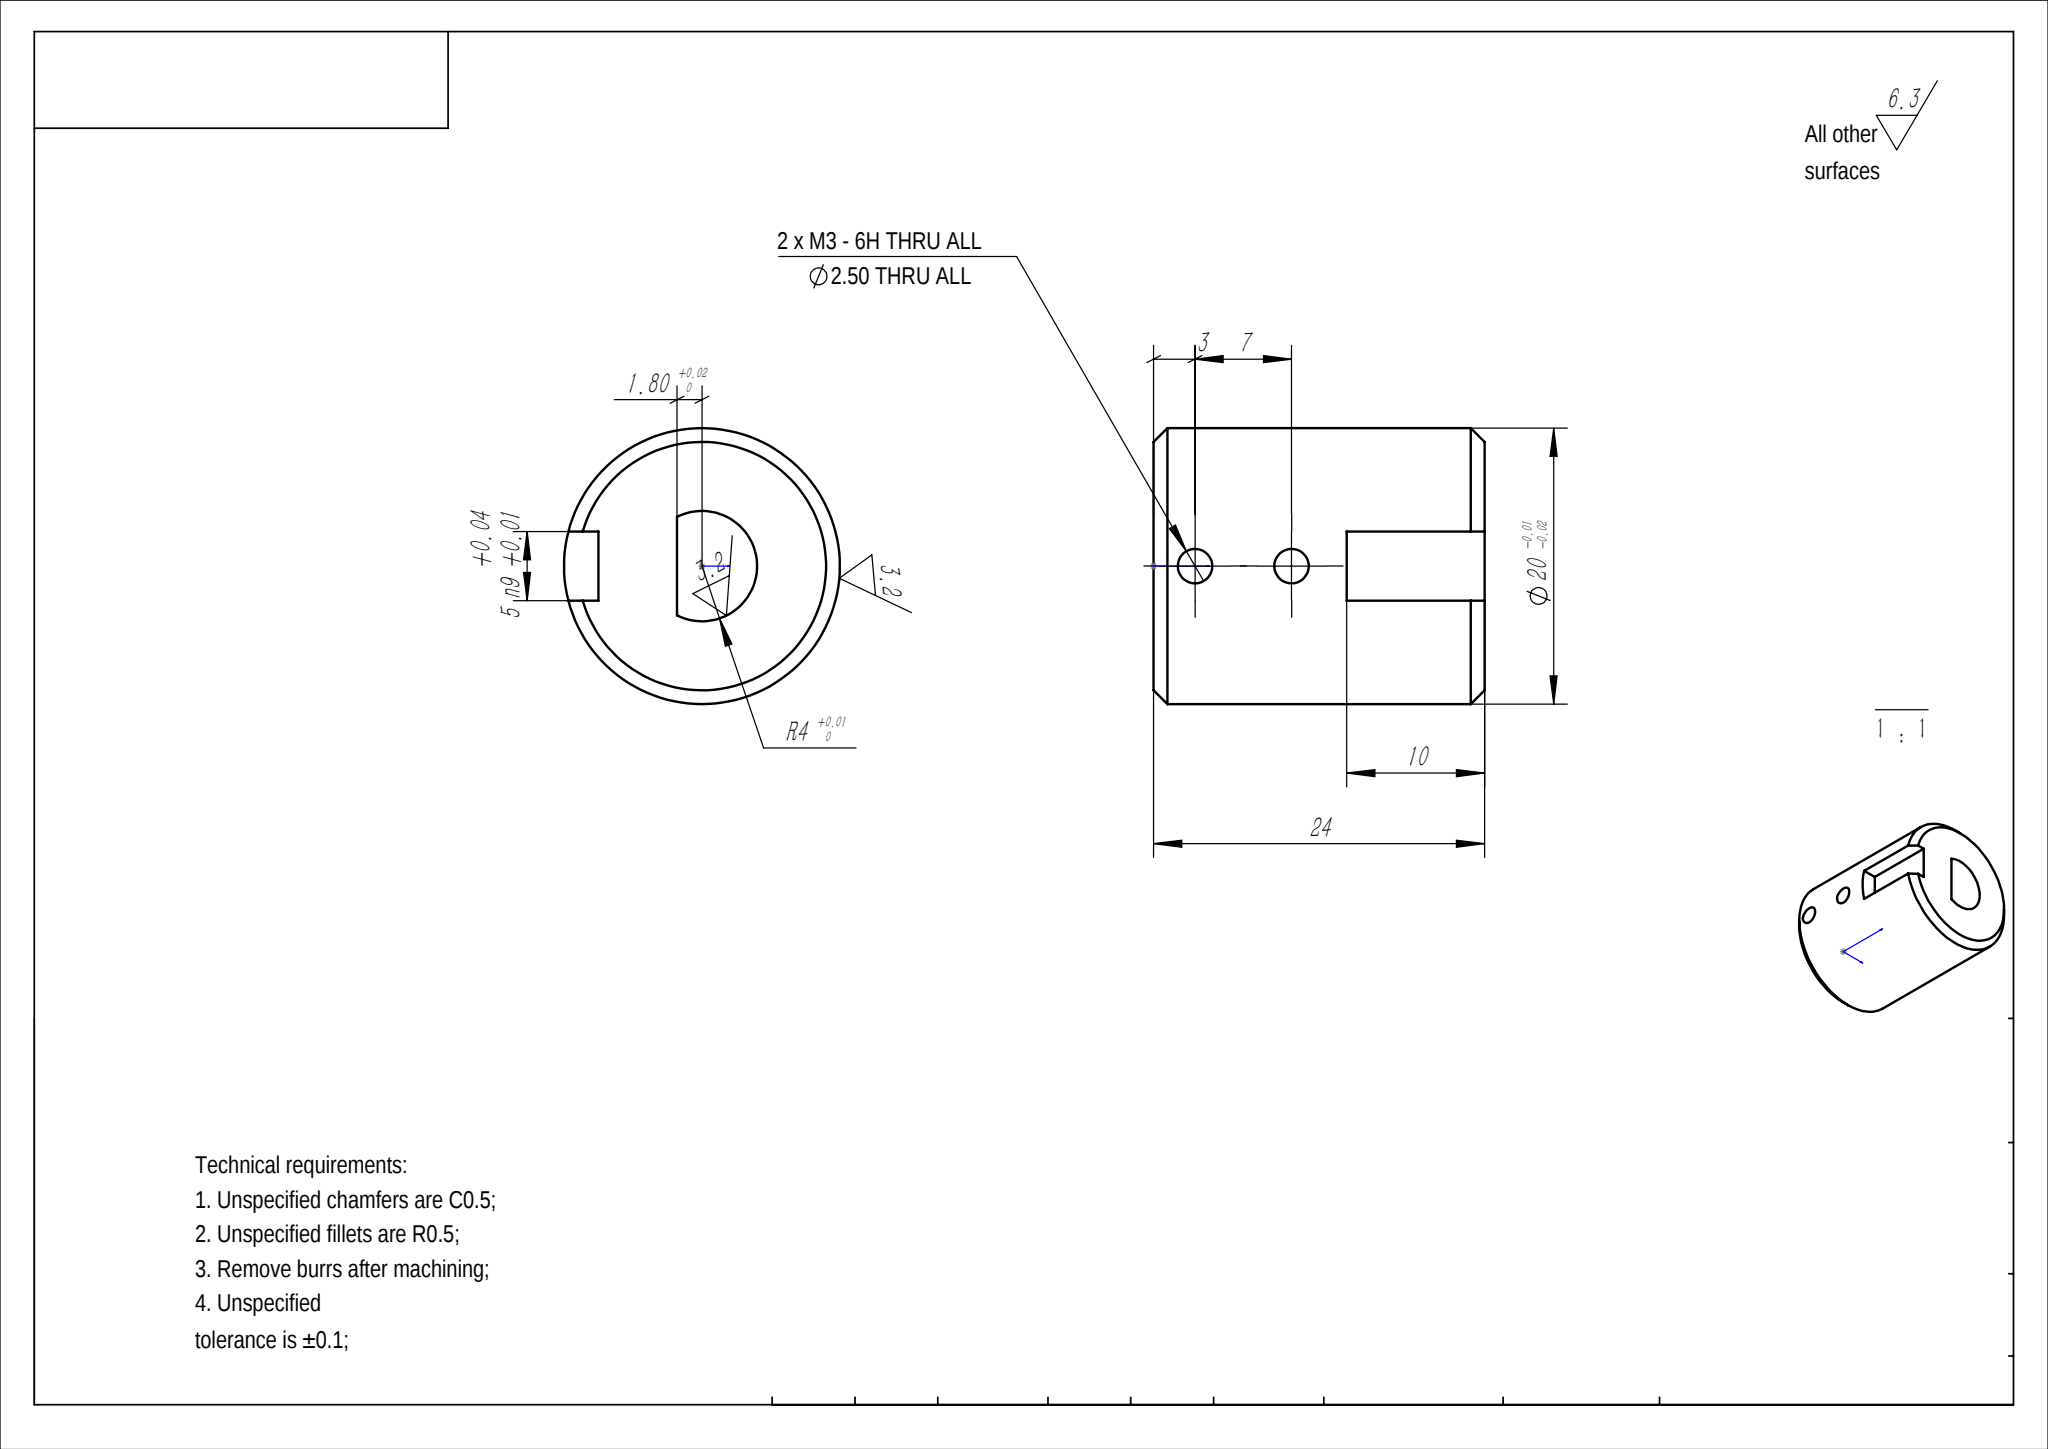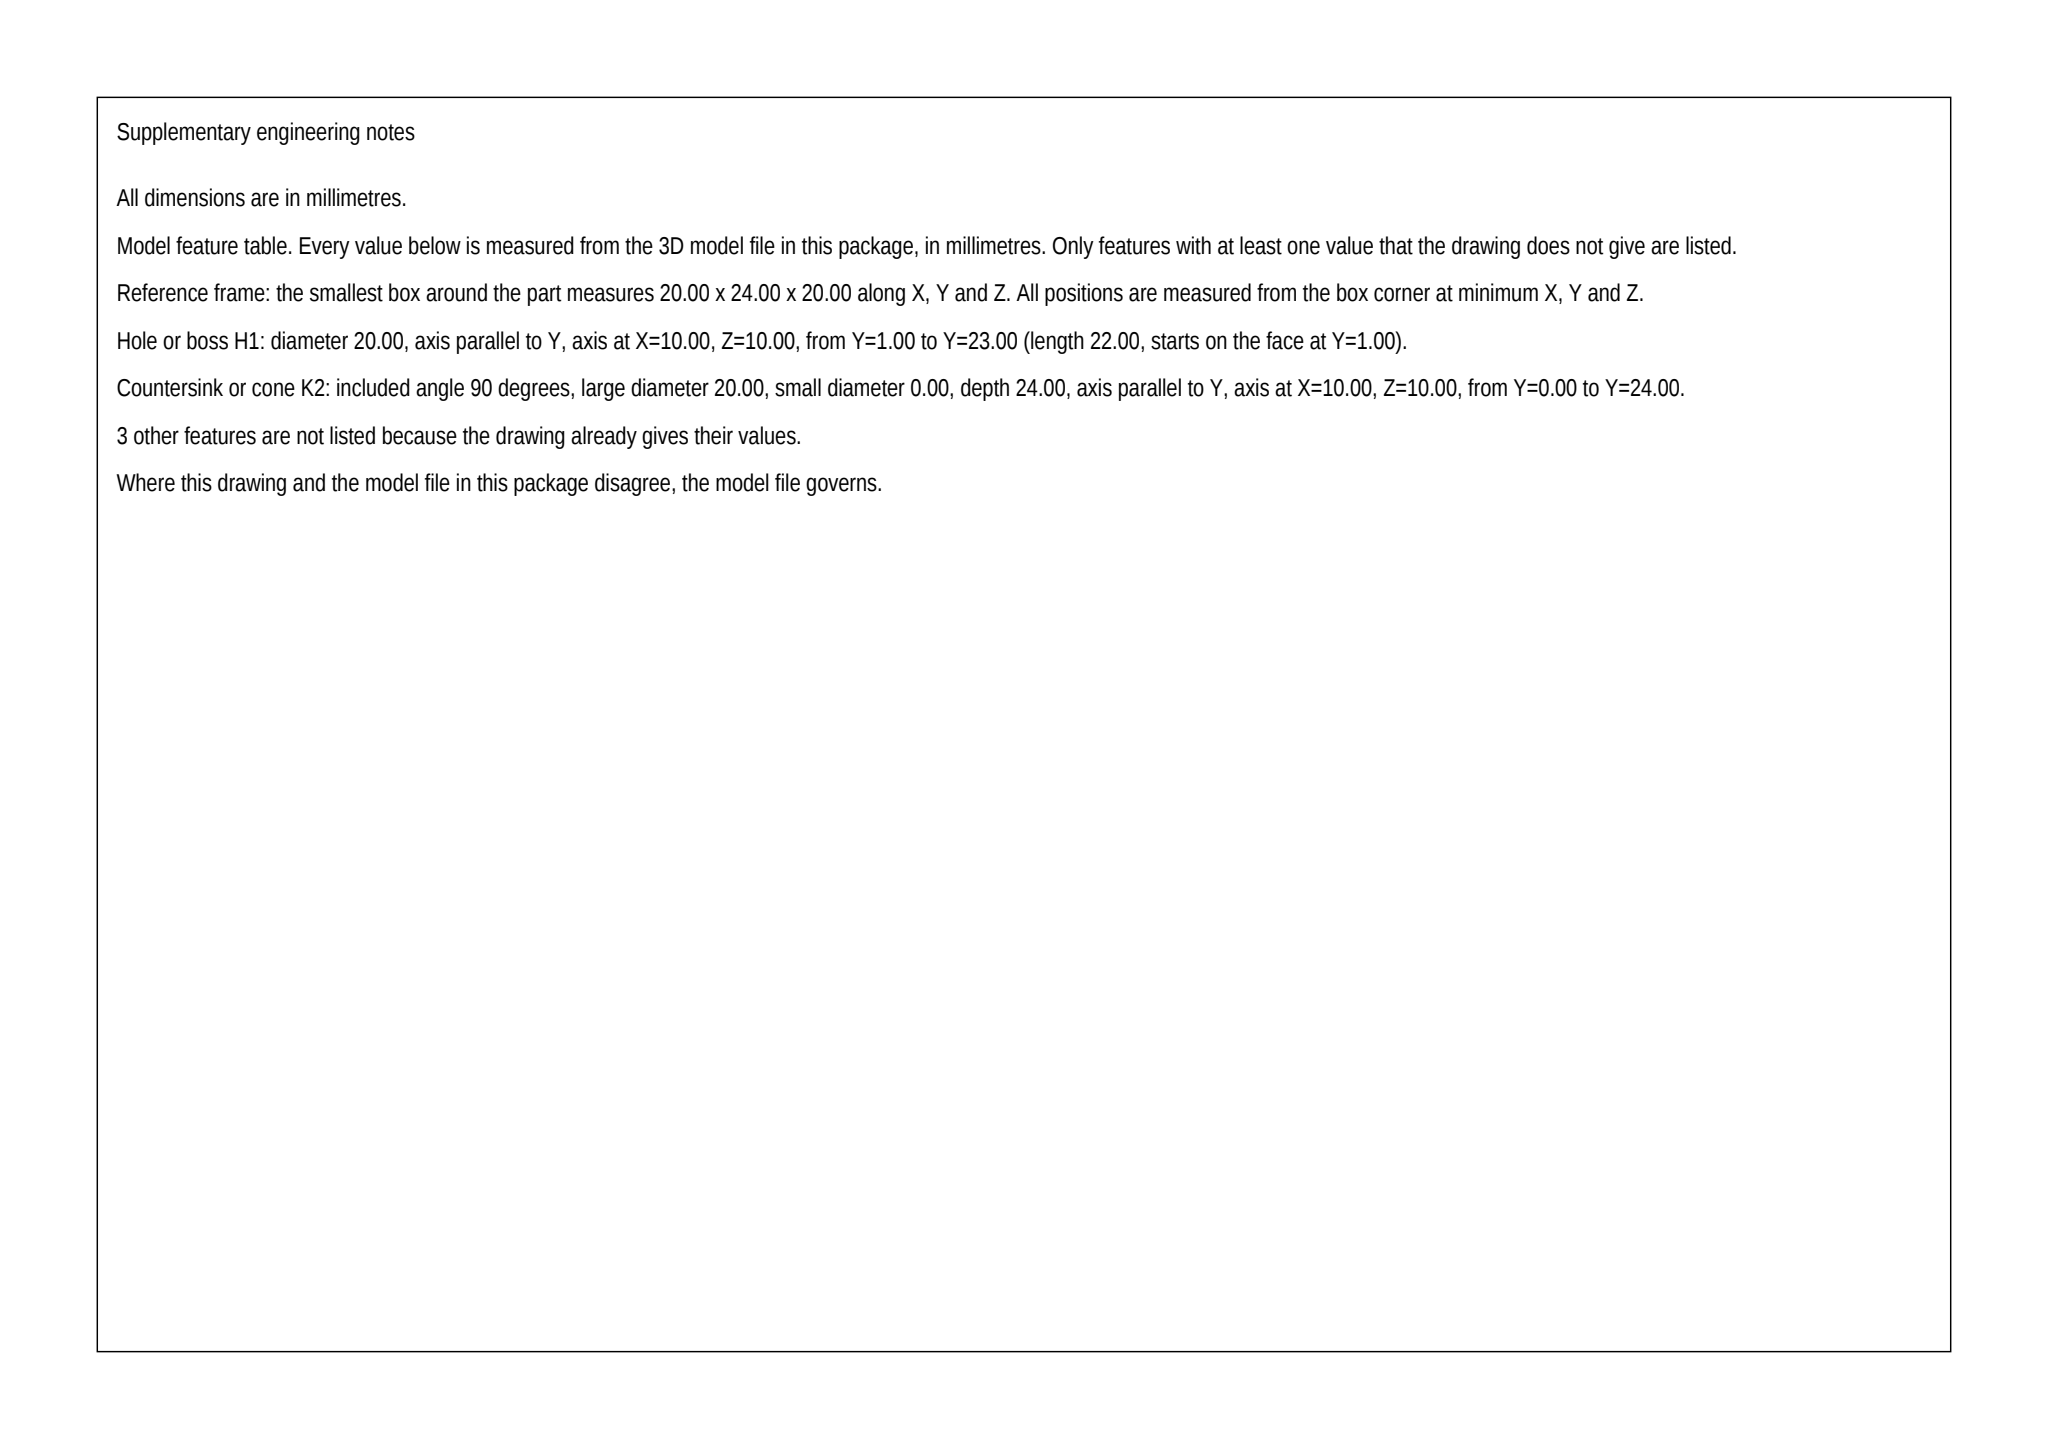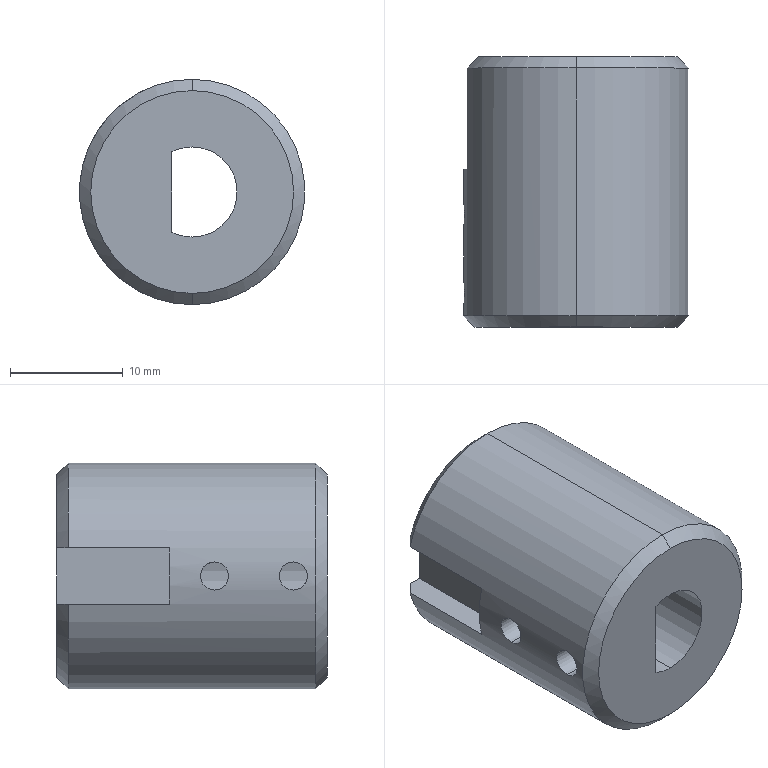Part | SolidWorks | mm | 1 solid | 21 faces | box 20 x 24 x 20 mm | volume 6345 mm3 | cylinder 9 | plane 7 | cone 5 | commonest cylinder face diameters 2.5 x4 8 x3 20 x2
build123d program:
from build123d import *

# Parameters (mm, degrees)
SKETCH1_R                  = 10
BOSS_EXTRUDE1_DEPTH        = 24
CUT_EXTRUDE1_DEPTH         = 30
SKETCH3_W                  = 1.25
SKETCH3_H                  = 8.2
M3_TAPPED_HOLE1_AT_2_COUNT = 2
M3_TAPPED_HOLE1_AT_2_PITCH = 7
SKETCH5_W                  = 5
SKETCH5_H                  = 5
CUT_EXTRUDE2_DEPTH         = 10
CHAMFER1_SIZE              = 1


with BuildPart() as part:
    # Sketch1 → Boss-Extrude1 (new body)
    with BuildSketch(Plane(origin=(0, 0, 0), x_dir=(1, 0, 0), z_dir=(0, 1, 0))):
        with Locations(Location((0, 0, 0), (0, 0, 270))):
            Circle(SKETCH1_R)
    extrude(amount=BOSS_EXTRUDE1_DEPTH)

    # Sketch2 → Cut-Extrude1 (cut)
    with BuildSketch(Plane(origin=(0, 24, 0), x_dir=(1, 0, 0), z_dir=(0, 1, 0))):
        with BuildLine():
            Line((-1.8, 3.572), (-1.8, -3.572))
            ThreePointArc((-1.8, -3.572), (4, 0), (-1.8, 3.572))
        make_face()
    extrude(amount=-CUT_EXTRUDE1_DEPTH, mode=Mode.SUBTRACT)

    # Sketch3 → M3 Tapped Hole1 (revolve, cut)
    with BuildSketch(Plane(origin=(-1.8, 3, 0), x_dir=(0, 0, -1), z_dir=(0, 1, 0))):
        with Locations((0.625, 4.1)):
            Rectangle(SKETCH3_W, SKETCH3_H)
    m3_tapped_hole1 = revolve(axis=Axis((4.55, 3, 0), (-1, 0, 0)), mode=Mode.SUBTRACT)

    # M3 Tapped Hole1 at 2: M3 Tapped Hole1 ×2
    with Locations(*[(0, i * M3_TAPPED_HOLE1_AT_2_PITCH, 0) for i in range(1, M3_TAPPED_HOLE1_AT_2_COUNT)]):
        add(m3_tapped_hole1, mode=Mode.SUBTRACT)

    # Sketch5 → Cut-Extrude2 (cut)
    with BuildSketch(Plane(origin=(0, 24, 0), x_dir=(1, 0, 0), z_dir=(0, 1, 0))):
        with Locations((-10, 0)):
            Rectangle(SKETCH5_W, SKETCH5_H)
    extrude(amount=-CUT_EXTRUDE2_DEPTH, mode=Mode.SUBTRACT)

    # Chamfer1
    chamfer1_edges = [part.edges().sort_by_distance(p)[0] for p in [
        (0, 0, -10),
        (7.906, 24, -6.124),
    ]]
    chamfer(chamfer1_edges, length=CHAMFER1_SIZE)


solid = part.part
STEP:
#1=CARTESIAN_POINT('',(0.,24.,9.));
#2=VERTEX_POINT('',#1);
#3=CARTESIAN_POINT('',(0.,24.,-9.));
#4=VERTEX_POINT('',#3);
#5=CARTESIAN_POINT('',(0.,24.,0.));
#6=DIRECTION('',(0.,1.,0.));
#7=DIRECTION('',(0.,0.,1.));
#8=AXIS2_PLACEMENT_3D('',#5,#6,#7);
#9=CIRCLE('',#8,9.);
#10=EDGE_CURVE('',#2,#4,#9,.T.);
#11=ORIENTED_EDGE('',*,*,#10,.F.);
#12=CARTESIAN_POINT('',(0.,23.,10.));
#13=VERTEX_POINT('',#12);
#14=CARTESIAN_POINT('',(0.,24.,9.));
#15=DIRECTION('',(0.,-0.7071,0.7071));
#16=VECTOR('',#15,1000.);
#17=LINE('',#14,#16);
#18=EDGE_CURVE('',#2,#13,#17,.T.);
#19=ORIENTED_EDGE('',*,*,#18,.T.);
#20=CARTESIAN_POINT('',(0.,23.,-10.));
#21=VERTEX_POINT('',#20);
#22=CARTESIAN_POINT('',(0.,23.,0.));
#23=DIRECTION('',(0.,-1.,0.));
#24=DIRECTION('',(0.,0.,1.));
#25=AXIS2_PLACEMENT_3D('',#22,#23,#24);
#26=CIRCLE('',#25,10.);
#27=EDGE_CURVE('',#21,#13,#26,.T.);
#28=ORIENTED_EDGE('',*,*,#27,.F.);
#29=CARTESIAN_POINT('',(0.,24.,-9.));
#30=DIRECTION('',(0.,-0.7071,-0.7071));
#31=VECTOR('',#30,1000.);
#32=LINE('',#29,#31);
#33=EDGE_CURVE('',#4,#21,#32,.T.);
#34=ORIENTED_EDGE('',*,*,#33,.F.);
#35=EDGE_LOOP('',(#11,#19,#28,#34));
#36=FACE_OUTER_BOUND('',#35,.T.);
#37=CARTESIAN_POINT('',(0.,24.,0.));
#38=DIRECTION('',(0.,-1.,0.));
#39=DIRECTION('',(0.,0.,-1.));
#40=AXIS2_PLACEMENT_3D('',#37,#38,#39);
#41=CONICAL_SURFACE('',#40,9.,0.7854);
#42=ADVANCED_FACE('',(#36),#41,.T.);
#43=CARTESIAN_POINT('',(-8.646,24.,-2.5));
#44=VERTEX_POINT('',#43);
#45=CARTESIAN_POINT('',(0.,24.,0.));
#46=DIRECTION('',(0.,1.,0.));
#47=DIRECTION('',(0.,0.,1.));
#48=AXIS2_PLACEMENT_3D('',#45,#46,#47);
#49=CIRCLE('',#48,9.);
#50=EDGE_CURVE('',#4,#44,#49,.T.);
#51=ORIENTED_EDGE('',*,*,#50,.F.);
#52=ORIENTED_EDGE('',*,*,#33,.T.);
#53=CARTESIAN_POINT('',(-9.682,23.,-2.5));
#54=VERTEX_POINT('',#53);
#55=CARTESIAN_POINT('',(0.,23.,0.));
#56=DIRECTION('',(0.,-1.,0.));
#57=DIRECTION('',(0.,0.,1.));
#58=AXIS2_PLACEMENT_3D('',#55,#56,#57);
#59=CIRCLE('',#58,10.);
#60=EDGE_CURVE('',#54,#21,#59,.T.);
#61=ORIENTED_EDGE('',*,*,#60,.F.);
#62=CARTESIAN_POINT('',(-8.646,24.,-2.5));
#63=CARTESIAN_POINT('',(-8.992,23.667,-2.5));
#64=CARTESIAN_POINT('',(-9.338,23.334,-2.5));
#65=CARTESIAN_POINT('',(-9.682,23.,-2.5));
#66=B_SPLINE_CURVE_WITH_KNOTS('',3,(#62,#63,#64,#65),.UNSPECIFIED.,.F.,.F.,(4,4),(0.,0.00144),.UNSPECIFIED.);
#67=EDGE_CURVE('',#44,#54,#66,.T.);
#68=ORIENTED_EDGE('',*,*,#67,.F.);
#69=EDGE_LOOP('',(#51,#52,#61,#68));
#70=FACE_OUTER_BOUND('',#69,.T.);
#71=CARTESIAN_POINT('',(0.,24.,0.));
#72=DIRECTION('',(0.,-1.,0.));
#73=DIRECTION('',(0.,0.,-1.));
#74=AXIS2_PLACEMENT_3D('',#71,#72,#73);
#75=CONICAL_SURFACE('',#74,9.,0.7854);
#76=ADVANCED_FACE('',(#70),#75,.T.);
#77=CARTESIAN_POINT('',(0.,0.,-9.));
#78=VERTEX_POINT('',#77);
#79=CARTESIAN_POINT('',(0.,0.,9.));
#80=VERTEX_POINT('',#79);
#81=CARTESIAN_POINT('',(0.,0.,0.));
#82=DIRECTION('',(0.,-1.,0.));
#83=DIRECTION('',(0.,0.,1.));
#84=AXIS2_PLACEMENT_3D('',#81,#82,#83);
#85=CIRCLE('',#84,9.);
#86=EDGE_CURVE('',#78,#80,#85,.T.);
#87=ORIENTED_EDGE('',*,*,#86,.F.);
#88=CARTESIAN_POINT('',(0.,1.,-10.));
#89=VERTEX_POINT('',#88);
#90=CARTESIAN_POINT('',(0.,1.,-10.));
#91=DIRECTION('',(0.,0.7071,-0.7071));
#92=VECTOR('',#91,1000.);
#93=LINE('',#90,#92);
#94=EDGE_CURVE('',#78,#89,#93,.T.);
#95=ORIENTED_EDGE('',*,*,#94,.T.);
#96=CARTESIAN_POINT('',(0.,1.,10.));
#97=VERTEX_POINT('',#96);
#98=CARTESIAN_POINT('',(0.,1.,0.));
#99=DIRECTION('',(0.,1.,0.));
#100=DIRECTION('',(0.,0.,1.));
#101=AXIS2_PLACEMENT_3D('',#98,#99,#100);
#102=CIRCLE('',#101,10.);
#103=EDGE_CURVE('',#97,#89,#102,.T.);
#104=ORIENTED_EDGE('',*,*,#103,.F.);
#105=CARTESIAN_POINT('',(0.,1.,10.));
#106=DIRECTION('',(0.,0.7071,0.7071));
#107=VECTOR('',#106,1000.);
#108=LINE('',#105,#107);
#109=EDGE_CURVE('',#80,#97,#108,.T.);
#110=ORIENTED_EDGE('',*,*,#109,.F.);
#111=EDGE_LOOP('',(#87,#95,#104,#110));
#112=FACE_OUTER_BOUND('',#111,.T.);
#113=CARTESIAN_POINT('',(0.,1.,0.));
#114=DIRECTION('',(0.,1.,0.));
#115=DIRECTION('',(0.,0.,1.));
#116=AXIS2_PLACEMENT_3D('',#113,#114,#115);
#117=CONICAL_SURFACE('',#116,10.,0.7854);
#118=ADVANCED_FACE('',(#112),#117,.T.);
#119=CARTESIAN_POINT('',(-9.922,3.,1.25));
#120=VERTEX_POINT('',#119);
#121=CARTESIAN_POINT('',(-9.922,3.,-1.25));
#122=VERTEX_POINT('',#121);
#123=CARTESIAN_POINT('',(-9.922,3.,1.25));
#124=CARTESIAN_POINT('',(-9.922,2.835,1.25));
#125=CARTESIAN_POINT('',(-9.926,2.672,1.217));
#126=CARTESIAN_POINT('',(-9.94,2.37,1.092));
#127=CARTESIAN_POINT('',(-9.951,2.231,0.999));
#128=CARTESIAN_POINT('',(-9.971,2.001,0.7687));
#129=CARTESIAN_POINT('',(-9.981,1.908,0.6294));
#130=CARTESIAN_POINT('',(-9.996,1.783,0.3287));
#131=CARTESIAN_POINT('',(-10.,1.75,0.1644));
#132=CARTESIAN_POINT('',(-10.,1.75,-0.1662));
#133=CARTESIAN_POINT('',(-9.996,1.783,-0.3284));
#134=CARTESIAN_POINT('',(-9.981,1.909,-0.631));
#135=CARTESIAN_POINT('',(-9.971,2.002,-0.7695));
#136=CARTESIAN_POINT('',(-9.951,2.232,-0.9996));
#137=CARTESIAN_POINT('',(-9.94,2.371,-1.093));
#138=CARTESIAN_POINT('',(-9.926,2.672,-1.217));
#139=CARTESIAN_POINT('',(-9.922,2.837,-1.25));
#140=CARTESIAN_POINT('',(-9.922,3.,-1.25));
#141=B_SPLINE_CURVE_WITH_KNOTS('',3,(#123,#124,#125,#126,#127,#128,#129,#130,#131,#132,#133,#134,#135,#136,#137,#138,#139,#140),.UNSPECIFIED.,.F.,.F.,(4,2,2,2,2,2,2,2,4),(0.005868,0.006357,0.006846,0.007335,0.007824,0.008313,0.008802,0.00929,0.009779),.UNSPECIFIED.);
#142=EDGE_CURVE('',#120,#122,#141,.T.);
#143=ORIENTED_EDGE('',*,*,#142,.F.);
#144=CARTESIAN_POINT('',(-1.8,3.,1.25));
#145=VERTEX_POINT('',#144);
#146=CARTESIAN_POINT('',(-1.8,3.,1.25));
#147=DIRECTION('',(1.,0.,0.));
#148=VECTOR('',#147,1000.);
#149=LINE('',#146,#148);
#150=EDGE_CURVE('',#120,#145,#149,.T.);
#151=ORIENTED_EDGE('',*,*,#150,.T.);
#152=CARTESIAN_POINT('',(-1.8,3.,-1.25));
#153=VERTEX_POINT('',#152);
#154=CARTESIAN_POINT('',(-1.8,3.,-0.));
#155=DIRECTION('',(1.,0.,0.));
#156=DIRECTION('',(0.,0.,-1.));
#157=AXIS2_PLACEMENT_3D('',#154,#155,#156);
#158=CIRCLE('',#157,1.25);
#159=EDGE_CURVE('',#145,#153,#158,.T.);
#160=ORIENTED_EDGE('',*,*,#159,.T.);
#161=CARTESIAN_POINT('',(-1.8,3.,-1.25));
#162=DIRECTION('',(1.,0.,0.));
#163=VECTOR('',#162,1000.);
#164=LINE('',#161,#163);
#165=EDGE_CURVE('',#122,#153,#164,.T.);
#166=ORIENTED_EDGE('',*,*,#165,.F.);
#167=EDGE_LOOP('',(#143,#151,#160,#166));
#168=FACE_OUTER_BOUND('',#167,.T.);
#169=CARTESIAN_POINT('',(-1.8,3.,-0.));
#170=DIRECTION('',(1.,0.,0.));
#171=DIRECTION('',(0.,0.,-1.));
#172=AXIS2_PLACEMENT_3D('',#169,#170,#171);
#173=CYLINDRICAL_SURFACE('',#172,1.25);
#174=ADVANCED_FACE('',(#168),#173,.F.);
#175=CARTESIAN_POINT('',(-9.922,10.,1.25));
#176=VERTEX_POINT('',#175);
#177=CARTESIAN_POINT('',(-9.922,10.,-1.25));
#178=VERTEX_POINT('',#177);
#179=CARTESIAN_POINT('',(-9.922,10.,1.25));
#180=CARTESIAN_POINT('',(-9.922,9.835,1.25));
#181=CARTESIAN_POINT('',(-9.926,9.672,1.217));
#182=CARTESIAN_POINT('',(-9.94,9.37,1.092));
#183=CARTESIAN_POINT('',(-9.951,9.231,0.999));
#184=CARTESIAN_POINT('',(-9.971,9.001,0.7687));
#185=CARTESIAN_POINT('',(-9.981,8.908,0.6294));
#186=CARTESIAN_POINT('',(-9.996,8.783,0.3287));
#187=CARTESIAN_POINT('',(-10.,8.75,0.1644));
#188=CARTESIAN_POINT('',(-10.,8.75,-0.1662));
#189=CARTESIAN_POINT('',(-9.996,8.783,-0.3284));
#190=CARTESIAN_POINT('',(-9.981,8.909,-0.631));
#191=CARTESIAN_POINT('',(-9.971,9.002,-0.7695));
#192=CARTESIAN_POINT('',(-9.951,9.232,-0.9996));
#193=CARTESIAN_POINT('',(-9.94,9.371,-1.093));
#194=CARTESIAN_POINT('',(-9.926,9.672,-1.217));
#195=CARTESIAN_POINT('',(-9.922,9.837,-1.25));
#196=CARTESIAN_POINT('',(-9.922,10.,-1.25));
#197=B_SPLINE_CURVE_WITH_KNOTS('',3,(#179,#180,#181,#182,#183,#184,#185,#186,#187,#188,#189,#190,#191,#192,#193,#194,#195,#196),.UNSPECIFIED.,.F.,.F.,(4,2,2,2,2,2,2,2,4),(0.005868,0.006357,0.006846,0.007335,0.007824,0.008313,0.008802,0.00929,0.009779),.UNSPECIFIED.);
#198=EDGE_CURVE('',#176,#178,#197,.T.);
#199=ORIENTED_EDGE('',*,*,#198,.F.);
#200=CARTESIAN_POINT('',(-1.8,10.,1.25));
#201=VERTEX_POINT('',#200);
#202=CARTESIAN_POINT('',(-1.8,10.,1.25));
#203=DIRECTION('',(1.,0.,0.));
#204=VECTOR('',#203,1000.);
#205=LINE('',#202,#204);
#206=EDGE_CURVE('',#176,#201,#205,.T.);
#207=ORIENTED_EDGE('',*,*,#206,.T.);
#208=CARTESIAN_POINT('',(-1.8,10.,-1.25));
#209=VERTEX_POINT('',#208);
#210=CARTESIAN_POINT('',(-1.8,10.,0.));
#211=DIRECTION('',(1.,0.,0.));
#212=DIRECTION('',(0.,0.,-1.));
#213=AXIS2_PLACEMENT_3D('',#210,#211,#212);
#214=CIRCLE('',#213,1.25);
#215=EDGE_CURVE('',#201,#209,#214,.T.);
#216=ORIENTED_EDGE('',*,*,#215,.T.);
#217=CARTESIAN_POINT('',(-1.8,10.,-1.25));
#218=DIRECTION('',(1.,0.,0.));
#219=VECTOR('',#218,1000.);
#220=LINE('',#217,#219);
#221=EDGE_CURVE('',#178,#209,#220,.T.);
#222=ORIENTED_EDGE('',*,*,#221,.F.);
#223=EDGE_LOOP('',(#199,#207,#216,#222));
#224=FACE_OUTER_BOUND('',#223,.T.);
#225=CARTESIAN_POINT('',(-1.8,10.,0.));
#226=DIRECTION('',(1.,0.,0.));
#227=DIRECTION('',(0.,0.,-1.));
#228=AXIS2_PLACEMENT_3D('',#225,#226,#227);
#229=CYLINDRICAL_SURFACE('',#228,1.25);
#230=ADVANCED_FACE('',(#224),#229,.F.);
#231=CARTESIAN_POINT('',(0.,0.,-4.));
#232=VERTEX_POINT('',#231);
#233=CARTESIAN_POINT('',(-1.8,0.,-3.572));
#234=VERTEX_POINT('',#233);
#235=CARTESIAN_POINT('',(0.,0.,0.));
#236=DIRECTION('',(0.,1.,0.));
#237=DIRECTION('',(0.,0.,1.));
#238=AXIS2_PLACEMENT_3D('',#235,#236,#237);
#239=CIRCLE('',#238,4.);
#240=EDGE_CURVE('',#232,#234,#239,.T.);
#241=ORIENTED_EDGE('',*,*,#240,.F.);
#242=CARTESIAN_POINT('',(0.,24.,-4.));
#243=VERTEX_POINT('',#242);
#244=CARTESIAN_POINT('',(0.,-6.,-4.));
#245=DIRECTION('',(0.,1.,0.));
#246=VECTOR('',#245,1000.);
#247=LINE('',#244,#246);
#248=EDGE_CURVE('',#232,#243,#247,.T.);
#249=ORIENTED_EDGE('',*,*,#248,.T.);
#250=CARTESIAN_POINT('',(-1.8,24.,-3.572));
#251=VERTEX_POINT('',#250);
#252=CARTESIAN_POINT('',(0.,24.,0.));
#253=DIRECTION('',(0.,1.,0.));
#254=DIRECTION('',(0.,0.,1.));
#255=AXIS2_PLACEMENT_3D('',#252,#253,#254);
#256=CIRCLE('',#255,4.);
#257=EDGE_CURVE('',#243,#251,#256,.T.);
#258=ORIENTED_EDGE('',*,*,#257,.T.);
#259=CARTESIAN_POINT('',(-1.8,-6.,-3.572));
#260=DIRECTION('',(0.,1.,0.));
#261=VECTOR('',#260,1000.);
#262=LINE('',#259,#261);
#263=EDGE_CURVE('',#234,#251,#262,.T.);
#264=ORIENTED_EDGE('',*,*,#263,.F.);
#265=EDGE_LOOP('',(#241,#249,#258,#264));
#266=FACE_OUTER_BOUND('',#265,.T.);
#267=CARTESIAN_POINT('',(0.,-6.,0.));
#268=DIRECTION('',(0.,1.,0.));
#269=DIRECTION('',(0.,0.,1.));
#270=AXIS2_PLACEMENT_3D('',#267,#268,#269);
#271=CYLINDRICAL_SURFACE('',#270,4.);
#272=ADVANCED_FACE('',(#266),#271,.F.);
#273=ORIENTED_EDGE('',*,*,#248,.F.);
#274=CARTESIAN_POINT('',(0.,0.,4.));
#275=VERTEX_POINT('',#274);
#276=CARTESIAN_POINT('',(0.,0.,0.));
#277=DIRECTION('',(0.,1.,0.));
#278=DIRECTION('',(0.,0.,1.));
#279=AXIS2_PLACEMENT_3D('',#276,#277,#278);
#280=CIRCLE('',#279,4.);
#281=EDGE_CURVE('',#275,#232,#280,.T.);
#282=ORIENTED_EDGE('',*,*,#281,.F.);
#283=CARTESIAN_POINT('',(0.,24.,4.));
#284=VERTEX_POINT('',#283);
#285=CARTESIAN_POINT('',(0.,-6.,4.));
#286=DIRECTION('',(0.,1.,0.));
#287=VECTOR('',#286,1000.);
#288=LINE('',#285,#287);
#289=EDGE_CURVE('',#275,#284,#288,.T.);
#290=ORIENTED_EDGE('',*,*,#289,.T.);
#291=CARTESIAN_POINT('',(0.,24.,0.));
#292=DIRECTION('',(0.,1.,0.));
#293=DIRECTION('',(0.,0.,1.));
#294=AXIS2_PLACEMENT_3D('',#291,#292,#293);
#295=CIRCLE('',#294,4.);
#296=EDGE_CURVE('',#284,#243,#295,.T.);
#297=ORIENTED_EDGE('',*,*,#296,.T.);
#298=EDGE_LOOP('',(#273,#282,#290,#297));
#299=FACE_OUTER_BOUND('',#298,.T.);
#300=CARTESIAN_POINT('',(0.,-6.,0.));
#301=DIRECTION('',(0.,1.,0.));
#302=DIRECTION('',(0.,0.,1.));
#303=AXIS2_PLACEMENT_3D('',#300,#301,#302);
#304=CYLINDRICAL_SURFACE('',#303,4.);
#305=ADVANCED_FACE('',(#299),#304,.F.);
#306=ORIENTED_EDGE('',*,*,#27,.T.);
#307=CARTESIAN_POINT('',(0.,24.,10.));
#308=DIRECTION('',(0.,-1.,0.));
#309=VECTOR('',#308,1000.);
#310=LINE('',#307,#309);
#311=EDGE_CURVE('',#13,#97,#310,.T.);
#312=ORIENTED_EDGE('',*,*,#311,.T.);
#313=ORIENTED_EDGE('',*,*,#103,.T.);
#314=CARTESIAN_POINT('',(0.,24.,-10.));
#315=DIRECTION('',(0.,-1.,0.));
#316=VECTOR('',#315,1000.);
#317=LINE('',#314,#316);
#318=EDGE_CURVE('',#21,#89,#317,.T.);
#319=ORIENTED_EDGE('',*,*,#318,.F.);
#320=EDGE_LOOP('',(#306,#312,#313,#319));
#321=FACE_OUTER_BOUND('',#320,.T.);
#322=CARTESIAN_POINT('',(0.,24.,0.));
#323=DIRECTION('',(0.,-1.,0.));
#324=DIRECTION('',(0.,0.,-1.));
#325=AXIS2_PLACEMENT_3D('',#322,#323,#324);
#326=CYLINDRICAL_SURFACE('',#325,10.);
#327=ADVANCED_FACE('',(#321),#326,.T.);
#328=ORIENTED_EDGE('',*,*,#311,.F.);
#329=CARTESIAN_POINT('',(-9.682,23.,2.5));
#330=VERTEX_POINT('',#329);
#331=CARTESIAN_POINT('',(0.,23.,0.));
#332=DIRECTION('',(0.,-1.,0.));
#333=DIRECTION('',(0.,0.,1.));
#334=AXIS2_PLACEMENT_3D('',#331,#332,#333);
#335=CIRCLE('',#334,10.);
#336=EDGE_CURVE('',#13,#330,#335,.T.);
#337=ORIENTED_EDGE('',*,*,#336,.T.);
#338=CARTESIAN_POINT('',(-9.682,14.,2.5));
#339=VERTEX_POINT('',#338);
#340=CARTESIAN_POINT('',(-9.682,24.,2.5));
#341=DIRECTION('',(0.,-1.,0.));
#342=VECTOR('',#341,1000.);
#343=LINE('',#340,#342);
#344=EDGE_CURVE('',#330,#339,#343,.T.);
#345=ORIENTED_EDGE('',*,*,#344,.T.);
#346=CARTESIAN_POINT('',(-9.682,14.,-2.5));
#347=VERTEX_POINT('',#346);
#348=CARTESIAN_POINT('',(0.,14.,0.));
#349=DIRECTION('',(0.,1.,0.));
#350=DIRECTION('',(0.,0.,1.));
#351=AXIS2_PLACEMENT_3D('',#348,#349,#350);
#352=CIRCLE('',#351,10.);
#353=EDGE_CURVE('',#347,#339,#352,.T.);
#354=ORIENTED_EDGE('',*,*,#353,.F.);
#355=CARTESIAN_POINT('',(-9.682,24.,-2.5));
#356=DIRECTION('',(0.,1.,0.));
#357=VECTOR('',#356,1000.);
#358=LINE('',#355,#357);
#359=EDGE_CURVE('',#347,#54,#358,.T.);
#360=ORIENTED_EDGE('',*,*,#359,.T.);
#361=ORIENTED_EDGE('',*,*,#60,.T.);
#362=ORIENTED_EDGE('',*,*,#318,.T.);
#363=CARTESIAN_POINT('',(0.,1.,0.));
#364=DIRECTION('',(0.,1.,0.));
#365=DIRECTION('',(0.,0.,1.));
#366=AXIS2_PLACEMENT_3D('',#363,#364,#365);
#367=CIRCLE('',#366,10.);
#368=EDGE_CURVE('',#89,#97,#367,.T.);
#369=ORIENTED_EDGE('',*,*,#368,.T.);
#370=EDGE_LOOP('',(#328,#337,#345,#354,#360,#361,#362,#369));
#371=FACE_OUTER_BOUND('',#370,.T.);
#372=CARTESIAN_POINT('',(-9.922,3.,-1.25));
#373=CARTESIAN_POINT('',(-9.922,3.082,-1.25));
#374=CARTESIAN_POINT('',(-9.923,3.165,-1.242));
#375=CARTESIAN_POINT('',(-9.927,3.325,-1.21));
#376=CARTESIAN_POINT('',(-9.929,3.403,-1.186));
#377=CARTESIAN_POINT('',(-9.94,3.63,-1.092));
#378=CARTESIAN_POINT('',(-9.951,3.768,-1.));
#379=CARTESIAN_POINT('',(-9.971,4.001,-0.767));
#380=CARTESIAN_POINT('',(-9.981,4.092,-0.6294));
#381=CARTESIAN_POINT('',(-9.992,4.186,-0.4024));
#382=CARTESIAN_POINT('',(-9.995,4.21,-0.3245));
#383=CARTESIAN_POINT('',(-9.999,4.242,-0.1641));
#384=CARTESIAN_POINT('',(-10.,4.25,-0.08118));
#385=CARTESIAN_POINT('',(-10.,4.25,0.1637));
#386=CARTESIAN_POINT('',(-9.996,4.217,0.3283));
#387=CARTESIAN_POINT('',(-9.981,4.092,0.6292));
#388=CARTESIAN_POINT('',(-9.971,3.999,0.7685));
#389=CARTESIAN_POINT('',(-9.951,3.769,0.999));
#390=CARTESIAN_POINT('',(-9.94,3.63,1.092));
#391=CARTESIAN_POINT('',(-9.926,3.328,1.217));
#392=CARTESIAN_POINT('',(-9.922,3.165,1.25));
#393=CARTESIAN_POINT('',(-9.922,3.,1.25));
#394=B_SPLINE_CURVE_WITH_KNOTS('',3,(#372,#373,#374,#375,#376,#377,#378,#379,#380,#381,#382,#383,#384,#385,#386,#387,#388,#389,#390,#391,#392,#393),.UNSPECIFIED.,.F.,.F.,(4,2,2,2,2,2,2,2,2,2,4),(0.001956,0.002201,0.002445,0.002934,0.003423,0.003668,0.003912,0.004401,0.00489,0.005379,0.005868),.UNSPECIFIED.);
#395=EDGE_CURVE('',#122,#120,#394,.T.);
#396=ORIENTED_EDGE('',*,*,#395,.T.);
#397=ORIENTED_EDGE('',*,*,#142,.T.);
#398=EDGE_LOOP('',(#396,#397));
#399=FACE_BOUND('',#398,.T.);
#400=CARTESIAN_POINT('',(-9.922,10.,-1.25));
#401=CARTESIAN_POINT('',(-9.922,10.082,-1.25));
#402=CARTESIAN_POINT('',(-9.923,10.165,-1.242));
#403=CARTESIAN_POINT('',(-9.927,10.325,-1.21));
#404=CARTESIAN_POINT('',(-9.929,10.403,-1.186));
#405=CARTESIAN_POINT('',(-9.94,10.63,-1.092));
#406=CARTESIAN_POINT('',(-9.951,10.768,-1.));
#407=CARTESIAN_POINT('',(-9.971,11.001,-0.767));
#408=CARTESIAN_POINT('',(-9.981,11.092,-0.6294));
#409=CARTESIAN_POINT('',(-9.992,11.186,-0.4024));
#410=CARTESIAN_POINT('',(-9.995,11.21,-0.3245));
#411=CARTESIAN_POINT('',(-9.999,11.242,-0.1641));
#412=CARTESIAN_POINT('',(-10.,11.25,-0.08118));
#413=CARTESIAN_POINT('',(-10.,11.25,0.1637));
#414=CARTESIAN_POINT('',(-9.996,11.217,0.3283));
#415=CARTESIAN_POINT('',(-9.981,11.092,0.6292));
#416=CARTESIAN_POINT('',(-9.971,10.999,0.7685));
#417=CARTESIAN_POINT('',(-9.951,10.769,0.999));
#418=CARTESIAN_POINT('',(-9.94,10.63,1.092));
#419=CARTESIAN_POINT('',(-9.926,10.328,1.217));
#420=CARTESIAN_POINT('',(-9.922,10.165,1.25));
#421=CARTESIAN_POINT('',(-9.922,10.,1.25));
#422=B_SPLINE_CURVE_WITH_KNOTS('',3,(#400,#401,#402,#403,#404,#405,#406,#407,#408,#409,#410,#411,#412,#413,#414,#415,#416,#417,#418,#419,#420,#421),.UNSPECIFIED.,.F.,.F.,(4,2,2,2,2,2,2,2,2,2,4),(0.001956,0.002201,0.002445,0.002934,0.003423,0.003668,0.003912,0.004401,0.00489,0.005379,0.005868),.UNSPECIFIED.);
#423=EDGE_CURVE('',#178,#176,#422,.T.);
#424=ORIENTED_EDGE('',*,*,#423,.T.);
#425=ORIENTED_EDGE('',*,*,#198,.T.);
#426=EDGE_LOOP('',(#424,#425));
#427=FACE_BOUND('',#426,.T.);
#428=CARTESIAN_POINT('',(0.,24.,0.));
#429=DIRECTION('',(0.,-1.,0.));
#430=DIRECTION('',(0.,0.,-1.));
#431=AXIS2_PLACEMENT_3D('',#428,#429,#430);
#432=CYLINDRICAL_SURFACE('',#431,10.);
#433=ADVANCED_FACE('',(#371,#399,#427),#432,.T.);
#434=CARTESIAN_POINT('',(-8.646,24.,2.5));
#435=VERTEX_POINT('',#434);
#436=CARTESIAN_POINT('',(-7.5,24.,2.5));
#437=VERTEX_POINT('',#436);
#438=CARTESIAN_POINT('',(0.,24.,2.5));
#439=DIRECTION('',(1.,0.,0.));
#440=VECTOR('',#439,1000.);
#441=LINE('',#438,#440);
#442=EDGE_CURVE('',#435,#437,#441,.T.);
#443=ORIENTED_EDGE('',*,*,#442,.F.);
#444=CARTESIAN_POINT('',(0.,24.,0.));
#445=DIRECTION('',(0.,1.,0.));
#446=DIRECTION('',(0.,0.,1.));
#447=AXIS2_PLACEMENT_3D('',#444,#445,#446);
#448=CIRCLE('',#447,9.);
#449=EDGE_CURVE('',#435,#2,#448,.T.);
#450=ORIENTED_EDGE('',*,*,#449,.T.);
#451=ORIENTED_EDGE('',*,*,#10,.T.);
#452=ORIENTED_EDGE('',*,*,#50,.T.);
#453=CARTESIAN_POINT('',(-7.5,24.,-2.5));
#454=VERTEX_POINT('',#453);
#455=CARTESIAN_POINT('',(-12.5,24.,-2.5));
#456=DIRECTION('',(-1.,0.,0.));
#457=VECTOR('',#456,1000.);
#458=LINE('',#455,#457);
#459=EDGE_CURVE('',#454,#44,#458,.T.);
#460=ORIENTED_EDGE('',*,*,#459,.F.);
#461=CARTESIAN_POINT('',(-7.5,24.,-2.5));
#462=DIRECTION('',(-0.,0.,-1.));
#463=VECTOR('',#462,1000.);
#464=LINE('',#461,#463);
#465=EDGE_CURVE('',#437,#454,#464,.T.);
#466=ORIENTED_EDGE('',*,*,#465,.F.);
#467=EDGE_LOOP('',(#443,#450,#451,#452,#460,#466));
#468=FACE_OUTER_BOUND('',#467,.T.);
#469=CARTESIAN_POINT('',(-1.8,24.,3.572));
#470=VERTEX_POINT('',#469);
#471=CARTESIAN_POINT('',(0.,24.,0.));
#472=DIRECTION('',(0.,1.,0.));
#473=DIRECTION('',(0.,0.,1.));
#474=AXIS2_PLACEMENT_3D('',#471,#472,#473);
#475=CIRCLE('',#474,4.);
#476=EDGE_CURVE('',#470,#284,#475,.T.);
#477=ORIENTED_EDGE('',*,*,#476,.F.);
#478=CARTESIAN_POINT('',(-1.8,24.,-3.572));
#479=DIRECTION('',(0.,0.,1.));
#480=VECTOR('',#479,1000.);
#481=LINE('',#478,#480);
#482=EDGE_CURVE('',#251,#470,#481,.T.);
#483=ORIENTED_EDGE('',*,*,#482,.F.);
#484=ORIENTED_EDGE('',*,*,#257,.F.);
#485=ORIENTED_EDGE('',*,*,#296,.F.);
#486=EDGE_LOOP('',(#477,#483,#484,#485));
#487=FACE_BOUND('',#486,.T.);
#488=CARTESIAN_POINT('',(0.,24.,0.));
#489=DIRECTION('',(0.,1.,0.));
#490=DIRECTION('',(0.,0.,1.));
#491=AXIS2_PLACEMENT_3D('',#488,#489,#490);
#492=PLANE('',#491);
#493=ADVANCED_FACE('',(#468,#487),#492,.T.);
#494=CARTESIAN_POINT('',(0.,0.,0.));
#495=DIRECTION('',(0.,-1.,0.));
#496=DIRECTION('',(0.,0.,1.));
#497=AXIS2_PLACEMENT_3D('',#494,#495,#496);
#498=CIRCLE('',#497,9.);
#499=EDGE_CURVE('',#80,#78,#498,.T.);
#500=ORIENTED_EDGE('',*,*,#499,.T.);
#501=ORIENTED_EDGE('',*,*,#86,.T.);
#502=EDGE_LOOP('',(#500,#501));
#503=FACE_OUTER_BOUND('',#502,.T.);
#504=CARTESIAN_POINT('',(-1.8,0.,3.572));
#505=VERTEX_POINT('',#504);
#506=CARTESIAN_POINT('',(-1.8,0.,0.));
#507=DIRECTION('',(0.,0.,1.));
#508=VECTOR('',#507,1000.);
#509=LINE('',#506,#508);
#510=EDGE_CURVE('',#234,#505,#509,.T.);
#511=ORIENTED_EDGE('',*,*,#510,.T.);
#512=CARTESIAN_POINT('',(0.,0.,0.));
#513=DIRECTION('',(0.,1.,0.));
#514=DIRECTION('',(0.,0.,1.));
#515=AXIS2_PLACEMENT_3D('',#512,#513,#514);
#516=CIRCLE('',#515,4.);
#517=EDGE_CURVE('',#505,#275,#516,.T.);
#518=ORIENTED_EDGE('',*,*,#517,.T.);
#519=ORIENTED_EDGE('',*,*,#281,.T.);
#520=ORIENTED_EDGE('',*,*,#240,.T.);
#521=EDGE_LOOP('',(#511,#518,#519,#520));
#522=FACE_BOUND('',#521,.T.);
#523=CARTESIAN_POINT('',(0.,0.,0.));
#524=DIRECTION('',(0.,1.,0.));
#525=DIRECTION('',(0.,0.,1.));
#526=AXIS2_PLACEMENT_3D('',#523,#524,#525);
#527=PLANE('',#526);
#528=ADVANCED_FACE('',(#503,#522),#527,.F.);
#529=ORIENTED_EDGE('',*,*,#289,.F.);
#530=ORIENTED_EDGE('',*,*,#517,.F.);
#531=CARTESIAN_POINT('',(-1.8,-6.,3.572));
#532=DIRECTION('',(0.,1.,0.));
#533=VECTOR('',#532,1000.);
#534=LINE('',#531,#533);
#535=EDGE_CURVE('',#505,#470,#534,.T.);
#536=ORIENTED_EDGE('',*,*,#535,.T.);
#537=ORIENTED_EDGE('',*,*,#476,.T.);
#538=EDGE_LOOP('',(#529,#530,#536,#537));
#539=FACE_OUTER_BOUND('',#538,.T.);
#540=CARTESIAN_POINT('',(0.,-6.,0.));
#541=DIRECTION('',(0.,1.,0.));
#542=DIRECTION('',(0.,0.,1.));
#543=AXIS2_PLACEMENT_3D('',#540,#541,#542);
#544=CYLINDRICAL_SURFACE('',#543,4.);
#545=ADVANCED_FACE('',(#539),#544,.F.);
#546=CARTESIAN_POINT('',(-1.8,3.,-0.));
#547=DIRECTION('',(1.,0.,0.));
#548=DIRECTION('',(0.,0.,-1.));
#549=AXIS2_PLACEMENT_3D('',#546,#547,#548);
#550=CIRCLE('',#549,1.25);
#551=EDGE_CURVE('',#153,#145,#550,.T.);
#552=ORIENTED_EDGE('',*,*,#551,.F.);
#553=ORIENTED_EDGE('',*,*,#159,.F.);
#554=EDGE_LOOP('',(#552,#553));
#555=FACE_BOUND('',#554,.T.);
#556=CARTESIAN_POINT('',(-1.8,10.,0.));
#557=DIRECTION('',(1.,0.,0.));
#558=DIRECTION('',(0.,0.,-1.));
#559=AXIS2_PLACEMENT_3D('',#556,#557,#558);
#560=CIRCLE('',#559,1.25);
#561=EDGE_CURVE('',#209,#201,#560,.T.);
#562=ORIENTED_EDGE('',*,*,#561,.F.);
#563=ORIENTED_EDGE('',*,*,#215,.F.);
#564=EDGE_LOOP('',(#562,#563));
#565=FACE_BOUND('',#564,.T.);
#566=ORIENTED_EDGE('',*,*,#263,.T.);
#567=ORIENTED_EDGE('',*,*,#482,.T.);
#568=ORIENTED_EDGE('',*,*,#535,.F.);
#569=ORIENTED_EDGE('',*,*,#510,.F.);
#570=EDGE_LOOP('',(#566,#567,#568,#569));
#571=FACE_OUTER_BOUND('',#570,.T.);
#572=CARTESIAN_POINT('',(-1.8,-6.,-3.572));
#573=DIRECTION('',(-1.,0.,0.));
#574=DIRECTION('',(0.,0.,1.));
#575=AXIS2_PLACEMENT_3D('',#572,#573,#574);
#576=PLANE('',#575);
#577=ADVANCED_FACE('',(#555,#565,#571),#576,.F.);
#578=ORIENTED_EDGE('',*,*,#206,.F.);
#579=ORIENTED_EDGE('',*,*,#423,.F.);
#580=ORIENTED_EDGE('',*,*,#221,.T.);
#581=ORIENTED_EDGE('',*,*,#561,.T.);
#582=EDGE_LOOP('',(#578,#579,#580,#581));
#583=FACE_OUTER_BOUND('',#582,.T.);
#584=CARTESIAN_POINT('',(-1.8,10.,0.));
#585=DIRECTION('',(1.,0.,0.));
#586=DIRECTION('',(0.,0.,-1.));
#587=AXIS2_PLACEMENT_3D('',#584,#585,#586);
#588=CYLINDRICAL_SURFACE('',#587,1.25);
#589=ADVANCED_FACE('',(#583),#588,.F.);
#590=ORIENTED_EDGE('',*,*,#150,.F.);
#591=ORIENTED_EDGE('',*,*,#395,.F.);
#592=ORIENTED_EDGE('',*,*,#165,.T.);
#593=ORIENTED_EDGE('',*,*,#551,.T.);
#594=EDGE_LOOP('',(#590,#591,#592,#593));
#595=FACE_OUTER_BOUND('',#594,.T.);
#596=CARTESIAN_POINT('',(-1.8,3.,-0.));
#597=DIRECTION('',(1.,0.,0.));
#598=DIRECTION('',(0.,0.,-1.));
#599=AXIS2_PLACEMENT_3D('',#596,#597,#598);
#600=CYLINDRICAL_SURFACE('',#599,1.25);
#601=ADVANCED_FACE('',(#595),#600,.F.);
#602=ORIENTED_EDGE('',*,*,#353,.T.);
#603=CARTESIAN_POINT('',(-7.5,14.,2.5));
#604=VERTEX_POINT('',#603);
#605=CARTESIAN_POINT('',(-12.5,14.,2.5));
#606=DIRECTION('',(1.,0.,0.));
#607=VECTOR('',#606,1000.);
#608=LINE('',#605,#607);
#609=EDGE_CURVE('',#339,#604,#608,.T.);
#610=ORIENTED_EDGE('',*,*,#609,.T.);
#611=CARTESIAN_POINT('',(-7.5,14.,-2.5));
#612=VERTEX_POINT('',#611);
#613=CARTESIAN_POINT('',(-7.5,14.,-2.5));
#614=DIRECTION('',(-0.,0.,-1.));
#615=VECTOR('',#614,1000.);
#616=LINE('',#613,#615);
#617=EDGE_CURVE('',#604,#612,#616,.T.);
#618=ORIENTED_EDGE('',*,*,#617,.T.);
#619=CARTESIAN_POINT('',(-12.5,14.,-2.5));
#620=DIRECTION('',(-1.,0.,0.));
#621=VECTOR('',#620,1000.);
#622=LINE('',#619,#621);
#623=EDGE_CURVE('',#612,#347,#622,.T.);
#624=ORIENTED_EDGE('',*,*,#623,.T.);
#625=EDGE_LOOP('',(#602,#610,#618,#624));
#626=FACE_OUTER_BOUND('',#625,.T.);
#627=CARTESIAN_POINT('',(0.,14.,0.));
#628=DIRECTION('',(0.,1.,0.));
#629=DIRECTION('',(0.,0.,1.));
#630=AXIS2_PLACEMENT_3D('',#627,#628,#629);
#631=PLANE('',#630);
#632=ADVANCED_FACE('',(#626),#631,.T.);
#633=ORIENTED_EDGE('',*,*,#344,.F.);
#634=CARTESIAN_POINT('',(-9.682,23.,2.5));
#635=CARTESIAN_POINT('',(-9.338,23.334,2.5));
#636=CARTESIAN_POINT('',(-8.992,23.667,2.5));
#637=CARTESIAN_POINT('',(-8.646,24.,2.5));
#638=B_SPLINE_CURVE_WITH_KNOTS('',3,(#634,#635,#636,#637),.UNSPECIFIED.,.F.,.F.,(4,4),(0.,0.00144),.UNSPECIFIED.);
#639=EDGE_CURVE('',#330,#435,#638,.T.);
#640=ORIENTED_EDGE('',*,*,#639,.T.);
#641=ORIENTED_EDGE('',*,*,#442,.T.);
#642=CARTESIAN_POINT('',(-7.5,14.,2.5));
#643=DIRECTION('',(0.,1.,0.));
#644=VECTOR('',#643,1000.);
#645=LINE('',#642,#644);
#646=EDGE_CURVE('',#604,#437,#645,.T.);
#647=ORIENTED_EDGE('',*,*,#646,.F.);
#648=ORIENTED_EDGE('',*,*,#609,.F.);
#649=EDGE_LOOP('',(#633,#640,#641,#647,#648));
#650=FACE_OUTER_BOUND('',#649,.T.);
#651=CARTESIAN_POINT('',(-12.5,14.,2.5));
#652=DIRECTION('',(0.,0.,1.));
#653=DIRECTION('',(1.,0.,0.));
#654=AXIS2_PLACEMENT_3D('',#651,#652,#653);
#655=PLANE('',#654);
#656=ADVANCED_FACE('',(#650),#655,.F.);
#657=ORIENTED_EDGE('',*,*,#459,.T.);
#658=ORIENTED_EDGE('',*,*,#67,.T.);
#659=ORIENTED_EDGE('',*,*,#359,.F.);
#660=ORIENTED_EDGE('',*,*,#623,.F.);
#661=CARTESIAN_POINT('',(-7.5,14.,-2.5));
#662=DIRECTION('',(0.,1.,0.));
#663=VECTOR('',#662,1000.);
#664=LINE('',#661,#663);
#665=EDGE_CURVE('',#612,#454,#664,.T.);
#666=ORIENTED_EDGE('',*,*,#665,.T.);
#667=EDGE_LOOP('',(#657,#658,#659,#660,#666));
#668=FACE_OUTER_BOUND('',#667,.T.);
#669=CARTESIAN_POINT('',(-12.5,14.,-2.5));
#670=DIRECTION('',(0.,0.,-1.));
#671=DIRECTION('',(-1.,0.,0.));
#672=AXIS2_PLACEMENT_3D('',#669,#670,#671);
#673=PLANE('',#672);
#674=ADVANCED_FACE('',(#668),#673,.F.);
#675=ORIENTED_EDGE('',*,*,#465,.T.);
#676=ORIENTED_EDGE('',*,*,#665,.F.);
#677=ORIENTED_EDGE('',*,*,#617,.F.);
#678=ORIENTED_EDGE('',*,*,#646,.T.);
#679=EDGE_LOOP('',(#675,#676,#677,#678));
#680=FACE_OUTER_BOUND('',#679,.T.);
#681=CARTESIAN_POINT('',(-7.5,14.,-2.5));
#682=DIRECTION('',(1.,0.,-0.));
#683=DIRECTION('',(-0.,0.,-1.));
#684=AXIS2_PLACEMENT_3D('',#681,#682,#683);
#685=PLANE('',#684);
#686=ADVANCED_FACE('',(#680),#685,.F.);
#687=ORIENTED_EDGE('',*,*,#94,.F.);
#688=ORIENTED_EDGE('',*,*,#499,.F.);
#689=ORIENTED_EDGE('',*,*,#109,.T.);
#690=ORIENTED_EDGE('',*,*,#368,.F.);
#691=EDGE_LOOP('',(#687,#688,#689,#690));
#692=FACE_OUTER_BOUND('',#691,.T.);
#693=CARTESIAN_POINT('',(0.,1.,0.));
#694=DIRECTION('',(0.,1.,0.));
#695=DIRECTION('',(0.,0.,1.));
#696=AXIS2_PLACEMENT_3D('',#693,#694,#695);
#697=CONICAL_SURFACE('',#696,10.,0.7854);
#698=ADVANCED_FACE('',(#692),#697,.T.);
#699=ORIENTED_EDGE('',*,*,#18,.F.);
#700=ORIENTED_EDGE('',*,*,#449,.F.);
#701=ORIENTED_EDGE('',*,*,#639,.F.);
#702=ORIENTED_EDGE('',*,*,#336,.F.);
#703=EDGE_LOOP('',(#699,#700,#701,#702));
#704=FACE_OUTER_BOUND('',#703,.T.);
#705=CARTESIAN_POINT('',(0.,24.,0.));
#706=DIRECTION('',(0.,-1.,0.));
#707=DIRECTION('',(0.,0.,-1.));
#708=AXIS2_PLACEMENT_3D('',#705,#706,#707);
#709=CONICAL_SURFACE('',#708,9.,0.7854);
#710=ADVANCED_FACE('',(#704),#709,.T.);
#711=CLOSED_SHELL('',(#42,#76,#118,#174,#230,#272,#305,#327,#433,#493,#528,#545,#577,#589,#601,#632,#656,#674,#686,#698,#710));
#712=MANIFOLD_SOLID_BREP('',#711);
#713=CARTESIAN_POINT('',(0.,0.,0.));
#714=DIRECTION('',(0.,0.,1.));
#715=DIRECTION('',(1.,0.,0.));
#716=AXIS2_PLACEMENT_3D('',#713,#714,#715);
#717=(LENGTH_UNIT()NAMED_UNIT(*)SI_UNIT(.MILLI.,.METRE.));
#718=UNCERTAINTY_MEASURE_WITH_UNIT(LENGTH_MEASURE(0.00001),#717,'','');
#719=(NAMED_UNIT(*)PLANE_ANGLE_UNIT()SI_UNIT($,.RADIAN.));
#720=(NAMED_UNIT(*)SI_UNIT($,.STERADIAN.)SOLID_ANGLE_UNIT());
#721=(GEOMETRIC_REPRESENTATION_CONTEXT(3)GLOBAL_UNCERTAINTY_ASSIGNED_CONTEXT((#718))GLOBAL_UNIT_ASSIGNED_CONTEXT((#717,#719,#720))REPRESENTATION_CONTEXT('',''));
#722=ADVANCED_BREP_SHAPE_REPRESENTATION('',(#712,#716),#721);